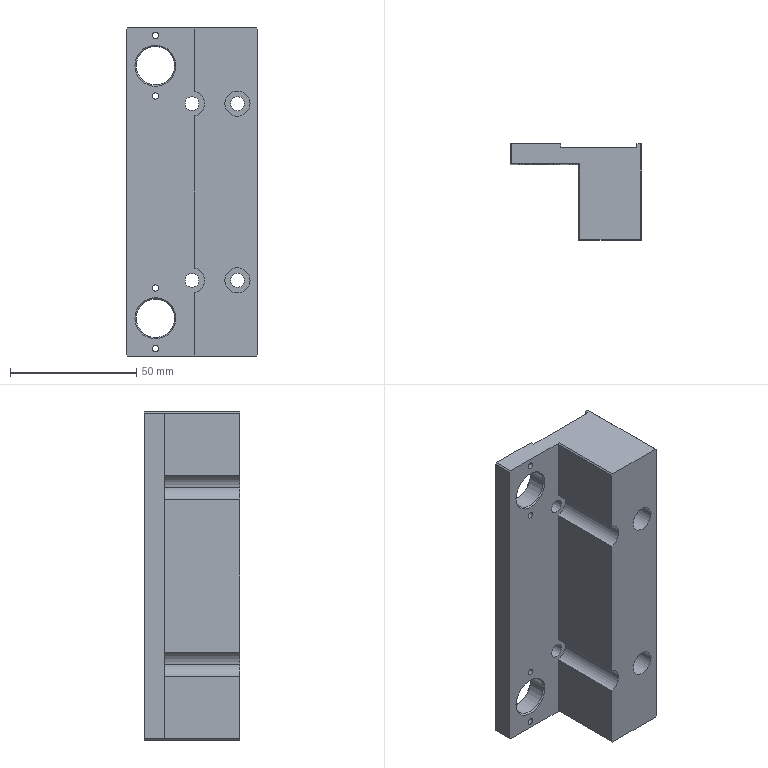Component | SolidWorks | LH-CGJ-01-057-1 | 1 solid | 58 faces | box 52 x 38 x 130 mm | volume 135497 mm3 | cylinder 28 | plane 22 | cone 8 | commonest cylinder face diameters 2.5 x8 10 x8 5.5 x8 15.2 x4 | material Black POM
build123d program:
from build123d import *

# Parameters (mm, degrees)
SKETCH1_W                                           = 130
SKETCH1_H                                           = 34
BOSS_EXTRUDE1_DEPTH                                 = 8
SKETCH2_W                                           = 30.2
SKETCH2_H                                           = 1.5
CUT_EXTRUDE1_DEPTH                                  = 135.611
SKETCH3_W                                           = 130
SKETCH3_H                                           = 25
BOSS_EXTRUDE2_DEPTH                                 = 30
SKETCH4_W                                           = 130
SKETCH4_H                                           = 8
BOSS_EXTRUDE3_DEPTH                                 = 18
SKETCH5_R                                           = 7.6
CUT_EXTRUDE2_DEPTH                                  = 10
CHAMFER1_SIZE                                       = 0.5
HOLE_SIZE_ACCORDING_TO_TYPE_1_OF_HEX_SO_D           = 5.5
HOLE_SIZE_ACCORDING_TO_TYPE_1_OF_HEX_SO_CBORE_D     = 10
HOLE_SIZE_ACCORDING_TO_TYPE_1_OF_HEX_SO_CBORE_DEPTH = 30
M3_TAPPED_HOLE1_D                                   = 2.5
LPATTERN1_COUNT                                     = 2
LPATTERN1_PITCH                                     = 100


with BuildPart() as part:
    # Sketch1 → Boss-Extrude1 (new body)
    with BuildSketch(Plane(origin=(0, 0, 0), x_dir=(1, 0, 0), z_dir=(0, 1, 0))):
        with Locations((65, 17)):
            Rectangle(SKETCH1_W, SKETCH1_H)
    extrude(amount=BOSS_EXTRUDE1_DEPTH)

    # Sketch2 → Cut-Extrude1 (cut, through all)
    with BuildSketch(Plane.ZY):
        with Locations((-17, 7.25)):
            Rectangle(SKETCH2_W, SKETCH2_H)
    extrude(amount=-CUT_EXTRUDE1_DEPTH, mode=Mode.SUBTRACT)

    # Sketch3 → Boss-Extrude2 (add)
    with BuildSketch(Plane.XZ):
        with Locations((65, -21.5)):
            Rectangle(SKETCH3_W, SKETCH3_H)
    extrude(amount=BOSS_EXTRUDE2_DEPTH)

    # Sketch4 → Boss-Extrude3 (add)
    with BuildSketch(Plane.XY):
        with Locations((65, 4)):
            Rectangle(SKETCH4_W, SKETCH4_H)
    extrude(amount=BOSS_EXTRUDE3_DEPTH)

    # Sketch5 → Cut-Extrude2 (cut)
    with BuildSketch(Plane.XZ):
        with Locations(Location((15, 6.5, 0), (0, 0, 270))):
            Circle(SKETCH5_R)
        with Locations(Location((115, 6.5, 0), (0, 0, 270))):
            Circle(SKETCH5_R)
    extrude(amount=-CUT_EXTRUDE2_DEPTH, mode=Mode.SUBTRACT)

    # Chamfer1
    chamfer1_edges = [part.edges().sort_by_distance(p)[0] for p in [
        (0, -15, -9),
        (130, -15, -9),
        (0, 4, 18),
        (130, 4, 18),
        (15, 8, 14.1),
        (15, 0, 14.1),
        (115, 8, 14.1),
        (115, 0, 14.1),
        (0, -11, -34),
        (130, -11, -34),
    ]]
    chamfer(chamfer1_edges, length=CHAMFER1_SIZE)

    # Hole Size_ according to_Type 1 of Hex So (through all)
    with Locations(Plane(origin=(0, -30, 0), x_dir=(-1, 0, 0), z_dir=(0, -1, 0))):
        with Locations((-30, 8), (-30, 26), (-100, 8), (-100, 26)):
            CounterBoreHole(HOLE_SIZE_ACCORDING_TO_TYPE_1_OF_HEX_SO_D / 2, HOLE_SIZE_ACCORDING_TO_TYPE_1_OF_HEX_SO_CBORE_D / 2, HOLE_SIZE_ACCORDING_TO_TYPE_1_OF_HEX_SO_CBORE_DEPTH)

    # M3 Tapped Hole1 (through all)
    with Locations(Plane(origin=(0, 0, 0), x_dir=(-1, 0, 0), z_dir=(0, -1, 0))):
        with Locations((-27, -6.5), (-3, -6.5)):
            m3_tapped_hole1 = Hole(M3_TAPPED_HOLE1_D / 2)

    # LPattern1: M3 Tapped Hole1 ×2
    with Locations(*[(i * LPATTERN1_PITCH, 0, 0) for i in range(1, LPATTERN1_COUNT)]):
        add(m3_tapped_hole1, mode=Mode.SUBTRACT)


solid = part.part

# Placed as in the assembly
solid = solid.moved(Location((-29.503, 21.715, 0.05), (0, -90, 0)))